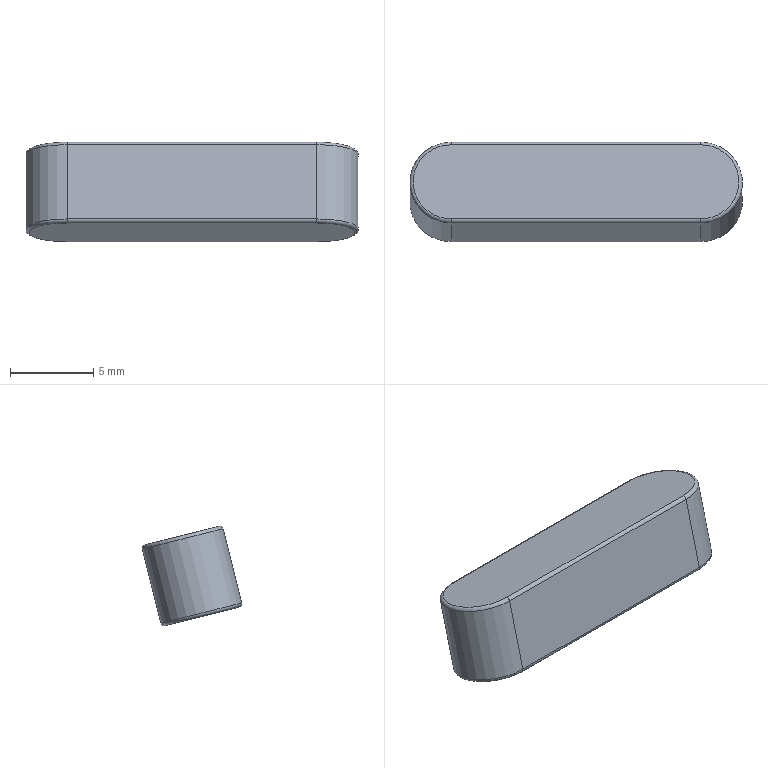Component | NX | STANDARD_FLAT_KEY_A_5X5X20 | 1 solid | 14 faces | box 20 x 5.98 x 5.98 mm | volume 472 mm3 | cylinder 6 | plane 4 | torus 4 | commonest cylinder face diameters 0.4 x4 5 x2
STEP:
#1=CARTESIAN_POINT('',(0.,0.,0.));
#2=DIRECTION('',(0.,0.,1.));
#3=DIRECTION('',(1.,0.,0.));
#4=AXIS2_PLACEMENT_3D('',#1,#2,#3);
#5=CARTESIAN_POINT('',(-38.948,64.186,69.841));
#6=VERTEX_POINT('',#5);
#7=CARTESIAN_POINT('',(-38.948,63.064,65.38));
#8=VERTEX_POINT('',#7);
#9=CARTESIAN_POINT('',(-38.948,64.235,70.035));
#10=DIRECTION('',(0.,-0.2438,-0.9698));
#11=VECTOR('',#10,1.);
#12=LINE('',#9,#11);
#13=CARTESIAN_POINT('',(-38.948,66.659,69.426));
#14=DIRECTION('',(0.,-0.2438,-0.9698));
#15=DIRECTION('',(1.,0.,0.));
#16=AXIS2_PLACEMENT_3D('',#13,#14,#15);
#17=CYLINDRICAL_SURFACE('',#16,2.5);
#18=CARTESIAN_POINT('',(1.571,0.));
#19=DIRECTION('',(0.,1.));
#20=VECTOR('',#19,1.);
#21=LINE('',#18,#20);
#22=(GEOMETRIC_REPRESENTATION_CONTEXT(2)PARAMETRIC_REPRESENTATION_CONTEXT()REPRESENTATION_CONTEXT('',''));
#23=DEFINITIONAL_REPRESENTATION('',(#21),#22);
#24=PCURVE('',#17,#23);
#25=CARTESIAN_POINT('',(-23.948,64.235,70.035));
#26=DIRECTION('',(-0.,-0.9698,0.2438));
#27=DIRECTION('',(-1.,0.,-0.));
#28=AXIS2_PLACEMENT_3D('',#25,#26,#27);
#29=PLANE('',#28);
#30=CARTESIAN_POINT('',(15.,-0.));
#31=DIRECTION('',(-0.,1.));
#32=VECTOR('',#31,1.);
#33=LINE('',#30,#32);
#34=(GEOMETRIC_REPRESENTATION_CONTEXT(2)PARAMETRIC_REPRESENTATION_CONTEXT()REPRESENTATION_CONTEXT('',''));
#35=DEFINITIONAL_REPRESENTATION('',(#33),#34);
#36=PCURVE('',#29,#35);
#37=SURFACE_CURVE('',#12,(#24,#36),.PCURVE_S1.);
#38=EDGE_CURVE('',#6,#8,#37,.T.);
#39=ORIENTED_EDGE('',*,*,#38,.F.);
#40=CARTESIAN_POINT('',(-38.948,69.035,68.622));
#41=VERTEX_POINT('',#40);
#42=CARTESIAN_POINT('',(-38.948,66.61,69.232));
#43=DIRECTION('',(0.,-0.2438,-0.9698));
#44=DIRECTION('',(1.,0.,0.));
#45=AXIS2_PLACEMENT_3D('',#42,#43,#44);
#46=CIRCLE('',#45,2.5);
#47=CARTESIAN_POINT('',(0.,0.2));
#48=DIRECTION('',(1.,-0.));
#49=VECTOR('',#48,1.);
#50=LINE('',#47,#49);
#51=(GEOMETRIC_REPRESENTATION_CONTEXT(2)PARAMETRIC_REPRESENTATION_CONTEXT()REPRESENTATION_CONTEXT('',''));
#52=DEFINITIONAL_REPRESENTATION('',(#50),#51);
#53=PCURVE('',#17,#52);
#54=CARTESIAN_POINT('',(-38.948,66.61,69.232));
#55=DIRECTION('',(0.,-0.2438,-0.9698));
#56=DIRECTION('',(1.,0.,0.));
#57=AXIS2_PLACEMENT_3D('',#54,#55,#56);
#58=TOROIDAL_SURFACE('',#57,2.3,0.2);
#59=CARTESIAN_POINT('',(0.,6.283));
#60=DIRECTION('',(1.,0.));
#61=VECTOR('',#60,1.);
#62=LINE('',#59,#61);
#63=(GEOMETRIC_REPRESENTATION_CONTEXT(2)PARAMETRIC_REPRESENTATION_CONTEXT()REPRESENTATION_CONTEXT('',''));
#64=DEFINITIONAL_REPRESENTATION('',(#62),#63);
#65=PCURVE('',#58,#64);
#66=SURFACE_CURVE('',#46,(#53,#65),.PCURVE_S1.);
#67=EDGE_CURVE('',#6,#41,#66,.T.);
#68=ORIENTED_EDGE('',*,*,#67,.T.);
#69=CARTESIAN_POINT('',(-38.948,67.914,64.161));
#70=VERTEX_POINT('',#69);
#71=CARTESIAN_POINT('',(-38.948,69.084,68.816));
#72=DIRECTION('',(0.,-0.2438,-0.9698));
#73=VECTOR('',#72,1.);
#74=LINE('',#71,#73);
#75=CARTESIAN_POINT('',(4.712,0.));
#76=DIRECTION('',(0.,1.));
#77=VECTOR('',#76,1.);
#78=LINE('',#75,#77);
#79=(GEOMETRIC_REPRESENTATION_CONTEXT(2)PARAMETRIC_REPRESENTATION_CONTEXT()REPRESENTATION_CONTEXT('',''));
#80=DEFINITIONAL_REPRESENTATION('',(#78),#79);
#81=PCURVE('',#17,#80);
#82=CARTESIAN_POINT('',(-38.948,69.084,68.816));
#83=DIRECTION('',(0.,0.9698,-0.2438));
#84=DIRECTION('',(0.,0.2438,0.9698));
#85=AXIS2_PLACEMENT_3D('',#82,#83,#84);
#86=PLANE('',#85);
#87=CARTESIAN_POINT('',(0.,0.));
#88=DIRECTION('',(-1.,0.));
#89=VECTOR('',#88,1.);
#90=LINE('',#87,#89);
#91=(GEOMETRIC_REPRESENTATION_CONTEXT(2)PARAMETRIC_REPRESENTATION_CONTEXT()REPRESENTATION_CONTEXT('',''));
#92=DEFINITIONAL_REPRESENTATION('',(#90),#91);
#93=PCURVE('',#86,#92);
#94=SURFACE_CURVE('',#74,(#81,#93),.PCURVE_S1.);
#95=EDGE_CURVE('',#41,#70,#94,.T.);
#96=ORIENTED_EDGE('',*,*,#95,.T.);
#97=CARTESIAN_POINT('',(-38.948,65.489,64.77));
#98=DIRECTION('',(0.,0.2438,0.9698));
#99=DIRECTION('',(1.,0.,0.));
#100=AXIS2_PLACEMENT_3D('',#97,#98,#99);
#101=CIRCLE('',#100,2.5);
#102=CARTESIAN_POINT('',(6.283,4.8));
#103=DIRECTION('',(-1.,0.));
#104=VECTOR('',#103,1.);
#105=LINE('',#102,#104);
#106=(GEOMETRIC_REPRESENTATION_CONTEXT(2)PARAMETRIC_REPRESENTATION_CONTEXT()REPRESENTATION_CONTEXT('',''));
#107=DEFINITIONAL_REPRESENTATION('',(#105),#106);
#108=PCURVE('',#17,#107);
#109=CARTESIAN_POINT('',(-38.948,65.489,64.77));
#110=DIRECTION('',(0.,-0.2438,-0.9698));
#111=DIRECTION('',(1.,0.,0.));
#112=AXIS2_PLACEMENT_3D('',#109,#110,#111);
#113=TOROIDAL_SURFACE('',#112,2.3,0.2);
#114=CARTESIAN_POINT('',(6.283,0.));
#115=DIRECTION('',(-1.,0.));
#116=VECTOR('',#115,1.);
#117=LINE('',#114,#116);
#118=(GEOMETRIC_REPRESENTATION_CONTEXT(2)PARAMETRIC_REPRESENTATION_CONTEXT()REPRESENTATION_CONTEXT('',''));
#119=DEFINITIONAL_REPRESENTATION('',(#117),#118);
#120=PCURVE('',#113,#119);
#121=SURFACE_CURVE('',#101,(#108,#120),.PCURVE_S1.);
#122=EDGE_CURVE('',#70,#8,#121,.T.);
#123=ORIENTED_EDGE('',*,*,#122,.T.);
#124=EDGE_LOOP('',(#39,#68,#96,#123));
#125=FACE_BOUND('',#124,.T.);
#126=ADVANCED_FACE('',(#125),#17,.T.);
#127=ORIENTED_EDGE('',*,*,#95,.F.);
#128=CARTESIAN_POINT('',(-23.948,69.035,68.622));
#129=VERTEX_POINT('',#128);
#130=CARTESIAN_POINT('',(-23.948,69.035,68.622));
#131=DIRECTION('',(1.,0.,0.));
#132=VECTOR('',#131,1.);
#133=LINE('',#130,#132);
#134=CARTESIAN_POINT('',(-0.2,15.));
#135=DIRECTION('',(0.,1.));
#136=VECTOR('',#135,1.);
#137=LINE('',#134,#136);
#138=(GEOMETRIC_REPRESENTATION_CONTEXT(2)PARAMETRIC_REPRESENTATION_CONTEXT()REPRESENTATION_CONTEXT('',''));
#139=DEFINITIONAL_REPRESENTATION('',(#137),#138);
#140=PCURVE('',#86,#139);
#141=CARTESIAN_POINT('',(-38.948,68.841,68.671));
#142=DIRECTION('',(-1.,0.,0.));
#143=DIRECTION('',(0.,-0.2438,-0.9698));
#144=AXIS2_PLACEMENT_3D('',#141,#142,#143);
#145=CYLINDRICAL_SURFACE('',#144,0.2);
#146=CARTESIAN_POINT('',(4.712,-15.));
#147=DIRECTION('',(0.,-1.));
#148=VECTOR('',#147,1.);
#149=LINE('',#146,#148);
#150=(GEOMETRIC_REPRESENTATION_CONTEXT(2)PARAMETRIC_REPRESENTATION_CONTEXT()REPRESENTATION_CONTEXT('',''));
#151=DEFINITIONAL_REPRESENTATION('',(#149),#150);
#152=PCURVE('',#145,#151);
#153=SURFACE_CURVE('',#133,(#140,#152),.PCURVE_S1.);
#154=EDGE_CURVE('',#41,#129,#153,.T.);
#155=ORIENTED_EDGE('',*,*,#154,.T.);
#156=CARTESIAN_POINT('',(-23.948,67.914,64.161));
#157=VERTEX_POINT('',#156);
#158=CARTESIAN_POINT('',(-23.948,69.084,68.816));
#159=DIRECTION('',(0.,-0.2438,-0.9698));
#160=VECTOR('',#159,1.);
#161=LINE('',#158,#160);
#162=CARTESIAN_POINT('',(0.,15.));
#163=DIRECTION('',(-1.,0.));
#164=VECTOR('',#163,1.);
#165=LINE('',#162,#164);
#166=(GEOMETRIC_REPRESENTATION_CONTEXT(2)PARAMETRIC_REPRESENTATION_CONTEXT()REPRESENTATION_CONTEXT('',''));
#167=DEFINITIONAL_REPRESENTATION('',(#165),#166);
#168=PCURVE('',#86,#167);
#169=CARTESIAN_POINT('',(-23.948,66.659,69.426));
#170=DIRECTION('',(0.,-0.2438,-0.9698));
#171=DIRECTION('',(1.,0.,0.));
#172=AXIS2_PLACEMENT_3D('',#169,#170,#171);
#173=CYLINDRICAL_SURFACE('',#172,2.5);
#174=CARTESIAN_POINT('',(4.712,0.));
#175=DIRECTION('',(0.,1.));
#176=VECTOR('',#175,1.);
#177=LINE('',#174,#176);
#178=(GEOMETRIC_REPRESENTATION_CONTEXT(2)PARAMETRIC_REPRESENTATION_CONTEXT()REPRESENTATION_CONTEXT('',''));
#179=DEFINITIONAL_REPRESENTATION('',(#177),#178);
#180=PCURVE('',#173,#179);
#181=SURFACE_CURVE('',#161,(#168,#180),.PCURVE_S1.);
#182=EDGE_CURVE('',#129,#157,#181,.T.);
#183=ORIENTED_EDGE('',*,*,#182,.T.);
#184=CARTESIAN_POINT('',(-38.948,67.914,64.161));
#185=DIRECTION('',(-1.,0.,0.));
#186=VECTOR('',#185,1.);
#187=LINE('',#184,#186);
#188=CARTESIAN_POINT('',(-4.8,0.));
#189=DIRECTION('',(0.,-1.));
#190=VECTOR('',#189,1.);
#191=LINE('',#188,#190);
#192=(GEOMETRIC_REPRESENTATION_CONTEXT(2)PARAMETRIC_REPRESENTATION_CONTEXT()REPRESENTATION_CONTEXT('',''));
#193=DEFINITIONAL_REPRESENTATION('',(#191),#192);
#194=PCURVE('',#86,#193);
#195=CARTESIAN_POINT('',(-38.948,67.72,64.21));
#196=DIRECTION('',(1.,0.,0.));
#197=DIRECTION('',(0.,0.2438,0.9698));
#198=AXIS2_PLACEMENT_3D('',#195,#196,#197);
#199=CYLINDRICAL_SURFACE('',#198,0.2);
#200=CARTESIAN_POINT('',(4.712,0.));
#201=DIRECTION('',(0.,-1.));
#202=VECTOR('',#201,1.);
#203=LINE('',#200,#202);
#204=(GEOMETRIC_REPRESENTATION_CONTEXT(2)PARAMETRIC_REPRESENTATION_CONTEXT()REPRESENTATION_CONTEXT('',''));
#205=DEFINITIONAL_REPRESENTATION('',(#203),#204);
#206=PCURVE('',#199,#205);
#207=SURFACE_CURVE('',#187,(#194,#206),.PCURVE_S1.);
#208=EDGE_CURVE('',#157,#70,#207,.T.);
#209=ORIENTED_EDGE('',*,*,#208,.T.);
#210=EDGE_LOOP('',(#127,#155,#183,#209));
#211=FACE_BOUND('',#210,.T.);
#212=ADVANCED_FACE('',(#211),#86,.T.);
#213=ORIENTED_EDGE('',*,*,#182,.F.);
#214=CARTESIAN_POINT('',(-23.948,64.186,69.841));
#215=VERTEX_POINT('',#214);
#216=CARTESIAN_POINT('',(-23.948,66.61,69.232));
#217=DIRECTION('',(0.,-0.2438,-0.9698));
#218=DIRECTION('',(1.,0.,0.));
#219=AXIS2_PLACEMENT_3D('',#216,#217,#218);
#220=CIRCLE('',#219,2.5);
#221=CARTESIAN_POINT('',(0.,0.2));
#222=DIRECTION('',(1.,0.));
#223=VECTOR('',#222,1.);
#224=LINE('',#221,#223);
#225=(GEOMETRIC_REPRESENTATION_CONTEXT(2)PARAMETRIC_REPRESENTATION_CONTEXT()REPRESENTATION_CONTEXT('',''));
#226=DEFINITIONAL_REPRESENTATION('',(#224),#225);
#227=PCURVE('',#173,#226);
#228=CARTESIAN_POINT('',(-23.948,66.61,69.232));
#229=DIRECTION('',(0.,-0.2438,-0.9698));
#230=DIRECTION('',(1.,0.,0.));
#231=AXIS2_PLACEMENT_3D('',#228,#229,#230);
#232=TOROIDAL_SURFACE('',#231,2.3,0.2);
#233=CARTESIAN_POINT('',(-0.,6.283));
#234=DIRECTION('',(1.,0.));
#235=VECTOR('',#234,1.);
#236=LINE('',#233,#235);
#237=(GEOMETRIC_REPRESENTATION_CONTEXT(2)PARAMETRIC_REPRESENTATION_CONTEXT()REPRESENTATION_CONTEXT('',''));
#238=DEFINITIONAL_REPRESENTATION('',(#236),#237);
#239=PCURVE('',#232,#238);
#240=SURFACE_CURVE('',#220,(#227,#239),.PCURVE_S1.);
#241=EDGE_CURVE('',#129,#215,#240,.T.);
#242=ORIENTED_EDGE('',*,*,#241,.T.);
#243=CARTESIAN_POINT('',(-23.948,63.064,65.38));
#244=VERTEX_POINT('',#243);
#245=CARTESIAN_POINT('',(-23.948,64.235,70.035));
#246=DIRECTION('',(0.,-0.2438,-0.9698));
#247=VECTOR('',#246,1.);
#248=LINE('',#245,#247);
#249=CARTESIAN_POINT('',(7.854,-0.));
#250=DIRECTION('',(0.,1.));
#251=VECTOR('',#250,1.);
#252=LINE('',#249,#251);
#253=(GEOMETRIC_REPRESENTATION_CONTEXT(2)PARAMETRIC_REPRESENTATION_CONTEXT()REPRESENTATION_CONTEXT('',''));
#254=DEFINITIONAL_REPRESENTATION('',(#252),#253);
#255=PCURVE('',#173,#254);
#256=CARTESIAN_POINT('',(-0.,-0.));
#257=DIRECTION('',(-0.,1.));
#258=VECTOR('',#257,1.);
#259=LINE('',#256,#258);
#260=(GEOMETRIC_REPRESENTATION_CONTEXT(2)PARAMETRIC_REPRESENTATION_CONTEXT()REPRESENTATION_CONTEXT('',''));
#261=DEFINITIONAL_REPRESENTATION('',(#259),#260);
#262=PCURVE('',#29,#261);
#263=SURFACE_CURVE('',#248,(#255,#262),.PCURVE_S1.);
#264=EDGE_CURVE('',#215,#244,#263,.T.);
#265=ORIENTED_EDGE('',*,*,#264,.T.);
#266=CARTESIAN_POINT('',(-23.948,65.489,64.77));
#267=DIRECTION('',(0.,0.2438,0.9698));
#268=DIRECTION('',(1.,0.,0.));
#269=AXIS2_PLACEMENT_3D('',#266,#267,#268);
#270=CIRCLE('',#269,2.5);
#271=CARTESIAN_POINT('',(12.566,4.8));
#272=DIRECTION('',(-1.,0.));
#273=VECTOR('',#272,1.);
#274=LINE('',#271,#273);
#275=(GEOMETRIC_REPRESENTATION_CONTEXT(2)PARAMETRIC_REPRESENTATION_CONTEXT()REPRESENTATION_CONTEXT('',''));
#276=DEFINITIONAL_REPRESENTATION('',(#274),#275);
#277=PCURVE('',#173,#276);
#278=CARTESIAN_POINT('',(-23.948,65.489,64.77));
#279=DIRECTION('',(0.,-0.2438,-0.9698));
#280=DIRECTION('',(1.,0.,0.));
#281=AXIS2_PLACEMENT_3D('',#278,#279,#280);
#282=TOROIDAL_SURFACE('',#281,2.3,0.2);
#283=CARTESIAN_POINT('',(12.566,0.));
#284=DIRECTION('',(-1.,0.));
#285=VECTOR('',#284,1.);
#286=LINE('',#283,#285);
#287=(GEOMETRIC_REPRESENTATION_CONTEXT(2)PARAMETRIC_REPRESENTATION_CONTEXT()REPRESENTATION_CONTEXT('',''));
#288=DEFINITIONAL_REPRESENTATION('',(#286),#287);
#289=PCURVE('',#282,#288);
#290=SURFACE_CURVE('',#270,(#277,#289),.PCURVE_S1.);
#291=EDGE_CURVE('',#244,#157,#290,.T.);
#292=ORIENTED_EDGE('',*,*,#291,.T.);
#293=EDGE_LOOP('',(#213,#242,#265,#292));
#294=FACE_BOUND('',#293,.T.);
#295=ADVANCED_FACE('',(#294),#173,.T.);
#296=ORIENTED_EDGE('',*,*,#264,.F.);
#297=CARTESIAN_POINT('',(-38.948,64.186,69.841));
#298=DIRECTION('',(-1.,0.,-0.));
#299=VECTOR('',#298,1.);
#300=LINE('',#297,#299);
#301=CARTESIAN_POINT('',(15.,0.2));
#302=DIRECTION('',(1.,0.));
#303=VECTOR('',#302,1.);
#304=LINE('',#301,#303);
#305=(GEOMETRIC_REPRESENTATION_CONTEXT(2)PARAMETRIC_REPRESENTATION_CONTEXT()REPRESENTATION_CONTEXT('',''));
#306=DEFINITIONAL_REPRESENTATION('',(#304),#305);
#307=PCURVE('',#29,#306);
#308=CARTESIAN_POINT('',(-23.948,64.38,69.792));
#309=DIRECTION('',(1.,-0.,0.));
#310=DIRECTION('',(-0.,-0.9698,0.2438));
#311=AXIS2_PLACEMENT_3D('',#308,#309,#310);
#312=CYLINDRICAL_SURFACE('',#311,0.2);
#313=CARTESIAN_POINT('',(6.283,-15.));
#314=DIRECTION('',(0.,-1.));
#315=VECTOR('',#314,1.);
#316=LINE('',#313,#315);
#317=(GEOMETRIC_REPRESENTATION_CONTEXT(2)PARAMETRIC_REPRESENTATION_CONTEXT()REPRESENTATION_CONTEXT('',''));
#318=DEFINITIONAL_REPRESENTATION('',(#316),#317);
#319=PCURVE('',#312,#318);
#320=SURFACE_CURVE('',#300,(#307,#319),.PCURVE_S1.);
#321=EDGE_CURVE('',#215,#6,#320,.T.);
#322=ORIENTED_EDGE('',*,*,#321,.T.);
#323=ORIENTED_EDGE('',*,*,#38,.T.);
#324=CARTESIAN_POINT('',(-23.948,63.064,65.38));
#325=DIRECTION('',(1.,-0.,0.));
#326=VECTOR('',#325,1.);
#327=LINE('',#324,#326);
#328=CARTESIAN_POINT('',(-0.,4.8));
#329=DIRECTION('',(-1.,-0.));
#330=VECTOR('',#329,1.);
#331=LINE('',#328,#330);
#332=(GEOMETRIC_REPRESENTATION_CONTEXT(2)PARAMETRIC_REPRESENTATION_CONTEXT()REPRESENTATION_CONTEXT('',''));
#333=DEFINITIONAL_REPRESENTATION('',(#331),#332);
#334=PCURVE('',#29,#333);
#335=CARTESIAN_POINT('',(-38.948,63.258,65.331));
#336=DIRECTION('',(-1.,0.,-0.));
#337=DIRECTION('',(0.,0.9698,-0.2438));
#338=AXIS2_PLACEMENT_3D('',#335,#336,#337);
#339=CYLINDRICAL_SURFACE('',#338,0.2);
#340=CARTESIAN_POINT('',(3.142,-15.));
#341=DIRECTION('',(0.,-1.));
#342=VECTOR('',#341,1.);
#343=LINE('',#340,#342);
#344=(GEOMETRIC_REPRESENTATION_CONTEXT(2)PARAMETRIC_REPRESENTATION_CONTEXT()REPRESENTATION_CONTEXT('',''));
#345=DEFINITIONAL_REPRESENTATION('',(#343),#344);
#346=PCURVE('',#339,#345);
#347=SURFACE_CURVE('',#327,(#334,#346),.PCURVE_S1.);
#348=EDGE_CURVE('',#8,#244,#347,.T.);
#349=ORIENTED_EDGE('',*,*,#348,.T.);
#350=EDGE_LOOP('',(#296,#322,#323,#349));
#351=FACE_BOUND('',#350,.T.);
#352=ADVANCED_FACE('',(#351),#29,.T.);
#353=CARTESIAN_POINT('',(-38.948,68.89,68.865));
#354=VERTEX_POINT('',#353);
#355=CARTESIAN_POINT('',(-38.948,64.429,69.986));
#356=VERTEX_POINT('',#355);
#357=CARTESIAN_POINT('',(-38.948,66.659,69.426));
#358=DIRECTION('',(0.,0.2438,0.9698));
#359=DIRECTION('',(1.,0.,0.));
#360=AXIS2_PLACEMENT_3D('',#357,#358,#359);
#361=CIRCLE('',#360,2.3);
#362=CARTESIAN_POINT('',(-38.948,66.659,69.426));
#363=DIRECTION('',(0.,-0.2438,-0.9698));
#364=DIRECTION('',(1.,0.,0.));
#365=AXIS2_PLACEMENT_3D('',#362,#363,#364);
#366=PLANE('',#365);
#367=CARTESIAN_POINT('',(2.3,0.));
#368=CARTESIAN_POINT('',(2.3,-3.984));
#369=CARTESIAN_POINT('',(-1.15,-1.992));
#370=CARTESIAN_POINT('',(-4.6,-0.));
#371=CARTESIAN_POINT('',(-1.15,1.992));
#372=CARTESIAN_POINT('',(2.3,3.984));
#373=CARTESIAN_POINT('',(2.3,0.));
#374=(BOUNDED_CURVE()B_SPLINE_CURVE(2,(#367,#368,#369,#370,#371,#372,#373),.UNSPECIFIED.,.T.,.F.)B_SPLINE_CURVE_WITH_KNOTS((1,2,2,2,2,1),(-2.094,0.,2.094,4.189,6.283,8.378),.UNSPECIFIED.)CURVE()GEOMETRIC_REPRESENTATION_ITEM()RATIONAL_B_SPLINE_CURVE((1.,0.5,1.,0.5,1.,0.5,1.))REPRESENTATION_ITEM(''));
#375=(GEOMETRIC_REPRESENTATION_CONTEXT(2)PARAMETRIC_REPRESENTATION_CONTEXT()REPRESENTATION_CONTEXT('',''));
#376=DEFINITIONAL_REPRESENTATION('',(#374),#375);
#377=PCURVE('',#366,#376);
#378=CARTESIAN_POINT('',(6.283,4.712));
#379=DIRECTION('',(-1.,0.));
#380=VECTOR('',#379,1.);
#381=LINE('',#378,#380);
#382=(GEOMETRIC_REPRESENTATION_CONTEXT(2)PARAMETRIC_REPRESENTATION_CONTEXT()REPRESENTATION_CONTEXT('',''));
#383=DEFINITIONAL_REPRESENTATION('',(#381),#382);
#384=PCURVE('',#58,#383);
#385=SURFACE_CURVE('',#361,(#377,#384),.PCURVE_S1.);
#386=EDGE_CURVE('',#354,#356,#385,.T.);
#387=ORIENTED_EDGE('',*,*,#386,.T.);
#388=CARTESIAN_POINT('',(-23.948,64.429,69.986));
#389=VERTEX_POINT('',#388);
#390=CARTESIAN_POINT('',(-23.948,64.429,69.986));
#391=DIRECTION('',(1.,-0.,0.));
#392=VECTOR('',#391,1.);
#393=LINE('',#390,#392);
#394=CARTESIAN_POINT('',(15.,2.3));
#395=DIRECTION('',(1.,0.));
#396=VECTOR('',#395,1.);
#397=LINE('',#394,#396);
#398=(GEOMETRIC_REPRESENTATION_CONTEXT(2)PARAMETRIC_REPRESENTATION_CONTEXT()REPRESENTATION_CONTEXT('',''));
#399=DEFINITIONAL_REPRESENTATION('',(#397),#398);
#400=PCURVE('',#366,#399);
#401=CARTESIAN_POINT('',(4.712,0.));
#402=DIRECTION('',(0.,1.));
#403=VECTOR('',#402,1.);
#404=LINE('',#401,#403);
#405=(GEOMETRIC_REPRESENTATION_CONTEXT(2)PARAMETRIC_REPRESENTATION_CONTEXT()REPRESENTATION_CONTEXT('',''));
#406=DEFINITIONAL_REPRESENTATION('',(#404),#405);
#407=PCURVE('',#312,#406);
#408=SURFACE_CURVE('',#393,(#400,#407),.PCURVE_S1.);
#409=EDGE_CURVE('',#356,#389,#408,.T.);
#410=ORIENTED_EDGE('',*,*,#409,.T.);
#411=CARTESIAN_POINT('',(-23.948,68.89,68.865));
#412=VERTEX_POINT('',#411);
#413=CARTESIAN_POINT('',(-23.948,66.659,69.426));
#414=DIRECTION('',(0.,0.2438,0.9698));
#415=DIRECTION('',(1.,0.,0.));
#416=AXIS2_PLACEMENT_3D('',#413,#414,#415);
#417=CIRCLE('',#416,2.3);
#418=CARTESIAN_POINT('',(17.3,0.));
#419=CARTESIAN_POINT('',(17.3,-3.984));
#420=CARTESIAN_POINT('',(13.85,-1.992));
#421=CARTESIAN_POINT('',(10.4,-0.));
#422=CARTESIAN_POINT('',(13.85,1.992));
#423=CARTESIAN_POINT('',(17.3,3.984));
#424=CARTESIAN_POINT('',(17.3,0.));
#425=(BOUNDED_CURVE()B_SPLINE_CURVE(2,(#418,#419,#420,#421,#422,#423,#424),.UNSPECIFIED.,.T.,.F.)B_SPLINE_CURVE_WITH_KNOTS((1,2,2,2,2,1),(-2.094,0.,2.094,4.189,6.283,8.378),.UNSPECIFIED.)CURVE()GEOMETRIC_REPRESENTATION_ITEM()RATIONAL_B_SPLINE_CURVE((1.,0.5,1.,0.5,1.,0.5,1.))REPRESENTATION_ITEM(''));
#426=(GEOMETRIC_REPRESENTATION_CONTEXT(2)PARAMETRIC_REPRESENTATION_CONTEXT()REPRESENTATION_CONTEXT('',''));
#427=DEFINITIONAL_REPRESENTATION('',(#425),#426);
#428=PCURVE('',#366,#427);
#429=CARTESIAN_POINT('',(12.566,4.712));
#430=DIRECTION('',(-1.,-0.));
#431=VECTOR('',#430,1.);
#432=LINE('',#429,#431);
#433=(GEOMETRIC_REPRESENTATION_CONTEXT(2)PARAMETRIC_REPRESENTATION_CONTEXT()REPRESENTATION_CONTEXT('',''));
#434=DEFINITIONAL_REPRESENTATION('',(#432),#433);
#435=PCURVE('',#232,#434);
#436=SURFACE_CURVE('',#417,(#428,#435),.PCURVE_S1.);
#437=EDGE_CURVE('',#389,#412,#436,.T.);
#438=ORIENTED_EDGE('',*,*,#437,.T.);
#439=CARTESIAN_POINT('',(-38.948,68.89,68.865));
#440=DIRECTION('',(-1.,0.,0.));
#441=VECTOR('',#440,1.);
#442=LINE('',#439,#441);
#443=CARTESIAN_POINT('',(0.,-2.3));
#444=DIRECTION('',(-1.,0.));
#445=VECTOR('',#444,1.);
#446=LINE('',#443,#445);
#447=(GEOMETRIC_REPRESENTATION_CONTEXT(2)PARAMETRIC_REPRESENTATION_CONTEXT()REPRESENTATION_CONTEXT('',''));
#448=DEFINITIONAL_REPRESENTATION('',(#446),#447);
#449=PCURVE('',#366,#448);
#450=CARTESIAN_POINT('',(3.142,0.));
#451=DIRECTION('',(0.,1.));
#452=VECTOR('',#451,1.);
#453=LINE('',#450,#452);
#454=(GEOMETRIC_REPRESENTATION_CONTEXT(2)PARAMETRIC_REPRESENTATION_CONTEXT()REPRESENTATION_CONTEXT('',''));
#455=DEFINITIONAL_REPRESENTATION('',(#453),#454);
#456=PCURVE('',#145,#455);
#457=SURFACE_CURVE('',#442,(#449,#456),.PCURVE_S1.);
#458=EDGE_CURVE('',#412,#354,#457,.T.);
#459=ORIENTED_EDGE('',*,*,#458,.T.);
#460=EDGE_LOOP('',(#387,#410,#438,#459));
#461=FACE_BOUND('',#460,.T.);
#462=ADVANCED_FACE('',(#461),#366,.F.);
#463=CARTESIAN_POINT('',(-23.948,67.671,64.016));
#464=VERTEX_POINT('',#463);
#465=CARTESIAN_POINT('',(-23.948,63.21,65.137));
#466=VERTEX_POINT('',#465);
#467=CARTESIAN_POINT('',(-23.948,65.44,64.577));
#468=DIRECTION('',(0.,-0.2438,-0.9698));
#469=DIRECTION('',(1.,0.,0.));
#470=AXIS2_PLACEMENT_3D('',#467,#468,#469);
#471=CIRCLE('',#470,2.3);
#472=CARTESIAN_POINT('',(-38.948,65.44,64.577));
#473=DIRECTION('',(0.,-0.2438,-0.9698));
#474=DIRECTION('',(1.,0.,0.));
#475=AXIS2_PLACEMENT_3D('',#472,#473,#474);
#476=PLANE('',#475);
#477=CARTESIAN_POINT('',(15.,0.));
#478=DIRECTION('',(1.,0.));
#479=AXIS2_PLACEMENT_2D('',#477,#478);
#480=CIRCLE('',#479,2.3);
#481=(GEOMETRIC_REPRESENTATION_CONTEXT(2)PARAMETRIC_REPRESENTATION_CONTEXT()REPRESENTATION_CONTEXT('',''));
#482=DEFINITIONAL_REPRESENTATION('',(#480),#481);
#483=PCURVE('',#476,#482);
#484=CARTESIAN_POINT('',(0.,1.571));
#485=DIRECTION('',(1.,-0.));
#486=VECTOR('',#485,1.);
#487=LINE('',#484,#486);
#488=(GEOMETRIC_REPRESENTATION_CONTEXT(2)PARAMETRIC_REPRESENTATION_CONTEXT()REPRESENTATION_CONTEXT('',''));
#489=DEFINITIONAL_REPRESENTATION('',(#487),#488);
#490=PCURVE('',#282,#489);
#491=SURFACE_CURVE('',#471,(#483,#490),.PCURVE_S1.);
#492=EDGE_CURVE('',#464,#466,#491,.T.);
#493=ORIENTED_EDGE('',*,*,#492,.T.);
#494=CARTESIAN_POINT('',(-38.948,63.21,65.137));
#495=VERTEX_POINT('',#494);
#496=CARTESIAN_POINT('',(-38.948,63.21,65.137));
#497=DIRECTION('',(-1.,0.,-0.));
#498=VECTOR('',#497,1.);
#499=LINE('',#496,#498);
#500=CARTESIAN_POINT('',(0.,2.3));
#501=DIRECTION('',(-1.,-0.));
#502=VECTOR('',#501,1.);
#503=LINE('',#500,#502);
#504=(GEOMETRIC_REPRESENTATION_CONTEXT(2)PARAMETRIC_REPRESENTATION_CONTEXT()REPRESENTATION_CONTEXT('',''));
#505=DEFINITIONAL_REPRESENTATION('',(#503),#504);
#506=PCURVE('',#476,#505);
#507=CARTESIAN_POINT('',(1.571,0.));
#508=DIRECTION('',(0.,1.));
#509=VECTOR('',#508,1.);
#510=LINE('',#507,#509);
#511=(GEOMETRIC_REPRESENTATION_CONTEXT(2)PARAMETRIC_REPRESENTATION_CONTEXT()REPRESENTATION_CONTEXT('',''));
#512=DEFINITIONAL_REPRESENTATION('',(#510),#511);
#513=PCURVE('',#339,#512);
#514=SURFACE_CURVE('',#499,(#506,#513),.PCURVE_S1.);
#515=EDGE_CURVE('',#466,#495,#514,.T.);
#516=ORIENTED_EDGE('',*,*,#515,.T.);
#517=CARTESIAN_POINT('',(-38.948,67.671,64.016));
#518=VERTEX_POINT('',#517);
#519=CARTESIAN_POINT('',(-38.948,65.44,64.577));
#520=DIRECTION('',(0.,-0.2438,-0.9698));
#521=DIRECTION('',(1.,0.,0.));
#522=AXIS2_PLACEMENT_3D('',#519,#520,#521);
#523=CIRCLE('',#522,2.3);
#524=CARTESIAN_POINT('',(0.,0.));
#525=DIRECTION('',(1.,0.));
#526=AXIS2_PLACEMENT_2D('',#524,#525);
#527=CIRCLE('',#526,2.3);
#528=(GEOMETRIC_REPRESENTATION_CONTEXT(2)PARAMETRIC_REPRESENTATION_CONTEXT()REPRESENTATION_CONTEXT('',''));
#529=DEFINITIONAL_REPRESENTATION('',(#527),#528);
#530=PCURVE('',#476,#529);
#531=CARTESIAN_POINT('',(0.,1.571));
#532=DIRECTION('',(1.,0.));
#533=VECTOR('',#532,1.);
#534=LINE('',#531,#533);
#535=(GEOMETRIC_REPRESENTATION_CONTEXT(2)PARAMETRIC_REPRESENTATION_CONTEXT()REPRESENTATION_CONTEXT('',''));
#536=DEFINITIONAL_REPRESENTATION('',(#534),#535);
#537=PCURVE('',#113,#536);
#538=SURFACE_CURVE('',#523,(#530,#537),.PCURVE_S1.);
#539=EDGE_CURVE('',#495,#518,#538,.T.);
#540=ORIENTED_EDGE('',*,*,#539,.T.);
#541=CARTESIAN_POINT('',(-38.948,67.671,64.016));
#542=DIRECTION('',(1.,0.,0.));
#543=VECTOR('',#542,1.);
#544=LINE('',#541,#543);
#545=CARTESIAN_POINT('',(0.,-2.3));
#546=DIRECTION('',(1.,0.));
#547=VECTOR('',#546,1.);
#548=LINE('',#545,#547);
#549=(GEOMETRIC_REPRESENTATION_CONTEXT(2)PARAMETRIC_REPRESENTATION_CONTEXT()REPRESENTATION_CONTEXT('',''));
#550=DEFINITIONAL_REPRESENTATION('',(#548),#549);
#551=PCURVE('',#476,#550);
#552=CARTESIAN_POINT('',(3.142,0.));
#553=DIRECTION('',(0.,1.));
#554=VECTOR('',#553,1.);
#555=LINE('',#552,#554);
#556=(GEOMETRIC_REPRESENTATION_CONTEXT(2)PARAMETRIC_REPRESENTATION_CONTEXT()REPRESENTATION_CONTEXT('',''));
#557=DEFINITIONAL_REPRESENTATION('',(#555),#556);
#558=PCURVE('',#199,#557);
#559=SURFACE_CURVE('',#544,(#551,#558),.PCURVE_S1.);
#560=EDGE_CURVE('',#518,#464,#559,.T.);
#561=ORIENTED_EDGE('',*,*,#560,.T.);
#562=EDGE_LOOP('',(#493,#516,#540,#561));
#563=FACE_BOUND('',#562,.T.);
#564=ADVANCED_FACE('',(#563),#476,.T.);
#565=CARTESIAN_POINT('',(-38.948,68.841,68.671));
#566=DIRECTION('',(-1.,0.,0.));
#567=DIRECTION('',(0.,-0.2438,-0.9698));
#568=AXIS2_PLACEMENT_3D('',#565,#566,#567);
#569=CIRCLE('',#568,0.2);
#570=CARTESIAN_POINT('',(0.,0.));
#571=DIRECTION('',(1.,0.));
#572=VECTOR('',#571,1.);
#573=LINE('',#570,#572);
#574=(GEOMETRIC_REPRESENTATION_CONTEXT(2)PARAMETRIC_REPRESENTATION_CONTEXT()REPRESENTATION_CONTEXT('',''));
#575=DEFINITIONAL_REPRESENTATION('',(#573),#574);
#576=PCURVE('',#145,#575);
#577=CARTESIAN_POINT('',(4.712,1.571));
#578=DIRECTION('',(0.,1.));
#579=VECTOR('',#578,1.);
#580=LINE('',#577,#579);
#581=(GEOMETRIC_REPRESENTATION_CONTEXT(2)PARAMETRIC_REPRESENTATION_CONTEXT()REPRESENTATION_CONTEXT('',''));
#582=DEFINITIONAL_REPRESENTATION('',(#580),#581);
#583=PCURVE('',#58,#582);
#584=SURFACE_CURVE('',#569,(#576,#583),.PCURVE_S1.);
#585=EDGE_CURVE('',#354,#41,#584,.T.);
#586=ORIENTED_EDGE('',*,*,#585,.F.);
#587=ORIENTED_EDGE('',*,*,#458,.F.);
#588=CARTESIAN_POINT('',(-23.948,68.841,68.671));
#589=DIRECTION('',(1.,-0.,-0.));
#590=DIRECTION('',(0.,0.2438,0.9698));
#591=AXIS2_PLACEMENT_3D('',#588,#589,#590);
#592=CIRCLE('',#591,0.2);
#593=CARTESIAN_POINT('',(9.425,-15.));
#594=DIRECTION('',(-1.,-0.));
#595=VECTOR('',#594,1.);
#596=LINE('',#593,#595);
#597=(GEOMETRIC_REPRESENTATION_CONTEXT(2)PARAMETRIC_REPRESENTATION_CONTEXT()REPRESENTATION_CONTEXT('',''));
#598=DEFINITIONAL_REPRESENTATION('',(#596),#597);
#599=PCURVE('',#145,#598);
#600=CARTESIAN_POINT('',(4.712,10.996));
#601=DIRECTION('',(-0.,-1.));
#602=VECTOR('',#601,1.);
#603=LINE('',#600,#602);
#604=(GEOMETRIC_REPRESENTATION_CONTEXT(2)PARAMETRIC_REPRESENTATION_CONTEXT()REPRESENTATION_CONTEXT('',''));
#605=DEFINITIONAL_REPRESENTATION('',(#603),#604);
#606=PCURVE('',#232,#605);
#607=SURFACE_CURVE('',#592,(#599,#606),.PCURVE_S1.);
#608=EDGE_CURVE('',#129,#412,#607,.T.);
#609=ORIENTED_EDGE('',*,*,#608,.F.);
#610=ORIENTED_EDGE('',*,*,#154,.F.);
#611=EDGE_LOOP('',(#586,#587,#609,#610));
#612=FACE_BOUND('',#611,.T.);
#613=ADVANCED_FACE('',(#612),#145,.T.);
#614=ORIENTED_EDGE('',*,*,#608,.T.);
#615=ORIENTED_EDGE('',*,*,#437,.F.);
#616=CARTESIAN_POINT('',(-23.948,64.38,69.792));
#617=DIRECTION('',(-1.,0.,0.));
#618=DIRECTION('',(-0.,-0.2438,-0.9698));
#619=AXIS2_PLACEMENT_3D('',#616,#617,#618);
#620=CIRCLE('',#619,0.2);
#621=CARTESIAN_POINT('',(7.854,7.854));
#622=DIRECTION('',(-0.,-1.));
#623=VECTOR('',#622,1.);
#624=LINE('',#621,#623);
#625=(GEOMETRIC_REPRESENTATION_CONTEXT(2)PARAMETRIC_REPRESENTATION_CONTEXT()REPRESENTATION_CONTEXT('',''));
#626=DEFINITIONAL_REPRESENTATION('',(#624),#625);
#627=PCURVE('',#232,#626);
#628=CARTESIAN_POINT('',(7.854,0.));
#629=DIRECTION('',(-1.,0.));
#630=VECTOR('',#629,1.);
#631=LINE('',#628,#630);
#632=(GEOMETRIC_REPRESENTATION_CONTEXT(2)PARAMETRIC_REPRESENTATION_CONTEXT()REPRESENTATION_CONTEXT('',''));
#633=DEFINITIONAL_REPRESENTATION('',(#631),#632);
#634=PCURVE('',#312,#633);
#635=SURFACE_CURVE('',#620,(#627,#634),.PCURVE_S1.);
#636=EDGE_CURVE('',#215,#389,#635,.T.);
#637=ORIENTED_EDGE('',*,*,#636,.F.);
#638=ORIENTED_EDGE('',*,*,#241,.F.);
#639=EDGE_LOOP('',(#614,#615,#637,#638));
#640=FACE_BOUND('',#639,.T.);
#641=ADVANCED_FACE('',(#640),#232,.T.);
#642=ORIENTED_EDGE('',*,*,#585,.T.);
#643=ORIENTED_EDGE('',*,*,#67,.F.);
#644=CARTESIAN_POINT('',(-38.948,64.38,69.792));
#645=DIRECTION('',(1.,-0.,0.));
#646=DIRECTION('',(-0.,-0.9698,0.2438));
#647=AXIS2_PLACEMENT_3D('',#644,#645,#646);
#648=CIRCLE('',#647,0.2);
#649=CARTESIAN_POINT('',(1.571,-0.));
#650=DIRECTION('',(0.,1.));
#651=VECTOR('',#650,1.);
#652=LINE('',#649,#651);
#653=(GEOMETRIC_REPRESENTATION_CONTEXT(2)PARAMETRIC_REPRESENTATION_CONTEXT()REPRESENTATION_CONTEXT('',''));
#654=DEFINITIONAL_REPRESENTATION('',(#652),#653);
#655=PCURVE('',#58,#654);
#656=CARTESIAN_POINT('',(0.,-15.));
#657=DIRECTION('',(1.,0.));
#658=VECTOR('',#657,1.);
#659=LINE('',#656,#658);
#660=(GEOMETRIC_REPRESENTATION_CONTEXT(2)PARAMETRIC_REPRESENTATION_CONTEXT()REPRESENTATION_CONTEXT('',''));
#661=DEFINITIONAL_REPRESENTATION('',(#659),#660);
#662=PCURVE('',#312,#661);
#663=SURFACE_CURVE('',#648,(#655,#662),.PCURVE_S1.);
#664=EDGE_CURVE('',#356,#6,#663,.T.);
#665=ORIENTED_EDGE('',*,*,#664,.F.);
#666=ORIENTED_EDGE('',*,*,#386,.F.);
#667=EDGE_LOOP('',(#642,#643,#665,#666));
#668=FACE_BOUND('',#667,.T.);
#669=ADVANCED_FACE('',(#668),#58,.T.);
#670=ORIENTED_EDGE('',*,*,#636,.T.);
#671=ORIENTED_EDGE('',*,*,#409,.F.);
#672=ORIENTED_EDGE('',*,*,#664,.T.);
#673=ORIENTED_EDGE('',*,*,#321,.F.);
#674=EDGE_LOOP('',(#670,#671,#672,#673));
#675=FACE_BOUND('',#674,.T.);
#676=ADVANCED_FACE('',(#675),#312,.T.);
#677=CARTESIAN_POINT('',(-38.948,67.72,64.21));
#678=DIRECTION('',(-1.,0.,0.));
#679=DIRECTION('',(0.,-0.2438,-0.9698));
#680=AXIS2_PLACEMENT_3D('',#677,#678,#679);
#681=CIRCLE('',#680,0.2);
#682=CARTESIAN_POINT('',(9.425,0.));
#683=DIRECTION('',(-1.,0.));
#684=VECTOR('',#683,1.);
#685=LINE('',#682,#684);
#686=(GEOMETRIC_REPRESENTATION_CONTEXT(2)PARAMETRIC_REPRESENTATION_CONTEXT()REPRESENTATION_CONTEXT('',''));
#687=DEFINITIONAL_REPRESENTATION('',(#685),#686);
#688=PCURVE('',#199,#687);
#689=CARTESIAN_POINT('',(4.712,-4.712));
#690=DIRECTION('',(0.,1.));
#691=VECTOR('',#690,1.);
#692=LINE('',#689,#691);
#693=(GEOMETRIC_REPRESENTATION_CONTEXT(2)PARAMETRIC_REPRESENTATION_CONTEXT()REPRESENTATION_CONTEXT('',''));
#694=DEFINITIONAL_REPRESENTATION('',(#692),#693);
#695=PCURVE('',#113,#694);
#696=SURFACE_CURVE('',#681,(#688,#695),.PCURVE_S1.);
#697=EDGE_CURVE('',#70,#518,#696,.T.);
#698=ORIENTED_EDGE('',*,*,#697,.F.);
#699=ORIENTED_EDGE('',*,*,#208,.F.);
#700=CARTESIAN_POINT('',(-23.948,67.72,64.21));
#701=DIRECTION('',(1.,0.,-0.));
#702=DIRECTION('',(0.,-0.9698,0.2438));
#703=AXIS2_PLACEMENT_3D('',#700,#701,#702);
#704=CIRCLE('',#703,0.2);
#705=CARTESIAN_POINT('',(1.571,15.));
#706=DIRECTION('',(1.,-0.));
#707=VECTOR('',#706,1.);
#708=LINE('',#705,#707);
#709=(GEOMETRIC_REPRESENTATION_CONTEXT(2)PARAMETRIC_REPRESENTATION_CONTEXT()REPRESENTATION_CONTEXT('',''));
#710=DEFINITIONAL_REPRESENTATION('',(#708),#709);
#711=PCURVE('',#199,#710);
#712=CARTESIAN_POINT('',(4.712,3.142));
#713=DIRECTION('',(-0.,-1.));
#714=VECTOR('',#713,1.);
#715=LINE('',#712,#714);
#716=(GEOMETRIC_REPRESENTATION_CONTEXT(2)PARAMETRIC_REPRESENTATION_CONTEXT()REPRESENTATION_CONTEXT('',''));
#717=DEFINITIONAL_REPRESENTATION('',(#715),#716);
#718=PCURVE('',#282,#717);
#719=SURFACE_CURVE('',#704,(#711,#718),.PCURVE_S1.);
#720=EDGE_CURVE('',#464,#157,#719,.T.);
#721=ORIENTED_EDGE('',*,*,#720,.F.);
#722=ORIENTED_EDGE('',*,*,#560,.F.);
#723=EDGE_LOOP('',(#698,#699,#721,#722));
#724=FACE_BOUND('',#723,.T.);
#725=ADVANCED_FACE('',(#724),#199,.T.);
#726=ORIENTED_EDGE('',*,*,#720,.T.);
#727=ORIENTED_EDGE('',*,*,#291,.F.);
#728=CARTESIAN_POINT('',(-23.948,63.258,65.331));
#729=DIRECTION('',(-1.,0.,-0.));
#730=DIRECTION('',(0.,0.9698,-0.2438));
#731=AXIS2_PLACEMENT_3D('',#728,#729,#730);
#732=CIRCLE('',#731,0.2);
#733=CARTESIAN_POINT('',(7.854,3.142));
#734=DIRECTION('',(0.,-1.));
#735=VECTOR('',#734,1.);
#736=LINE('',#733,#735);
#737=(GEOMETRIC_REPRESENTATION_CONTEXT(2)PARAMETRIC_REPRESENTATION_CONTEXT()REPRESENTATION_CONTEXT('',''));
#738=DEFINITIONAL_REPRESENTATION('',(#736),#737);
#739=PCURVE('',#282,#738);
#740=CARTESIAN_POINT('',(-0.,-15.));
#741=DIRECTION('',(1.,0.));
#742=VECTOR('',#741,1.);
#743=LINE('',#740,#742);
#744=(GEOMETRIC_REPRESENTATION_CONTEXT(2)PARAMETRIC_REPRESENTATION_CONTEXT()REPRESENTATION_CONTEXT('',''));
#745=DEFINITIONAL_REPRESENTATION('',(#743),#744);
#746=PCURVE('',#339,#745);
#747=SURFACE_CURVE('',#732,(#739,#746),.PCURVE_S1.);
#748=EDGE_CURVE('',#466,#244,#747,.T.);
#749=ORIENTED_EDGE('',*,*,#748,.F.);
#750=ORIENTED_EDGE('',*,*,#492,.F.);
#751=EDGE_LOOP('',(#726,#727,#749,#750));
#752=FACE_BOUND('',#751,.T.);
#753=ADVANCED_FACE('',(#752),#282,.T.);
#754=ORIENTED_EDGE('',*,*,#697,.T.);
#755=ORIENTED_EDGE('',*,*,#539,.F.);
#756=CARTESIAN_POINT('',(-38.948,63.258,65.331));
#757=DIRECTION('',(1.,0.,0.));
#758=DIRECTION('',(-0.,0.2438,0.9698));
#759=AXIS2_PLACEMENT_3D('',#756,#757,#758);
#760=CIRCLE('',#759,0.2);
#761=CARTESIAN_POINT('',(1.571,-1.571));
#762=DIRECTION('',(0.,1.));
#763=VECTOR('',#762,1.);
#764=LINE('',#761,#763);
#765=(GEOMETRIC_REPRESENTATION_CONTEXT(2)PARAMETRIC_REPRESENTATION_CONTEXT()REPRESENTATION_CONTEXT('',''));
#766=DEFINITIONAL_REPRESENTATION('',(#764),#765);
#767=PCURVE('',#113,#766);
#768=CARTESIAN_POINT('',(4.712,0.));
#769=DIRECTION('',(-1.,0.));
#770=VECTOR('',#769,1.);
#771=LINE('',#768,#770);
#772=(GEOMETRIC_REPRESENTATION_CONTEXT(2)PARAMETRIC_REPRESENTATION_CONTEXT()REPRESENTATION_CONTEXT('',''));
#773=DEFINITIONAL_REPRESENTATION('',(#771),#772);
#774=PCURVE('',#339,#773);
#775=SURFACE_CURVE('',#760,(#767,#774),.PCURVE_S1.);
#776=EDGE_CURVE('',#8,#495,#775,.T.);
#777=ORIENTED_EDGE('',*,*,#776,.F.);
#778=ORIENTED_EDGE('',*,*,#122,.F.);
#779=EDGE_LOOP('',(#754,#755,#777,#778));
#780=FACE_BOUND('',#779,.T.);
#781=ADVANCED_FACE('',(#780),#113,.T.);
#782=ORIENTED_EDGE('',*,*,#748,.T.);
#783=ORIENTED_EDGE('',*,*,#348,.F.);
#784=ORIENTED_EDGE('',*,*,#776,.T.);
#785=ORIENTED_EDGE('',*,*,#515,.F.);
#786=EDGE_LOOP('',(#782,#783,#784,#785));
#787=FACE_BOUND('',#786,.T.);
#788=ADVANCED_FACE('',(#787),#339,.T.);
#789=CLOSED_SHELL('',(#126,#212,#295,#352,#462,#564,#613,#641,#669,#676,#725,#753,#781,#788));
#790=MANIFOLD_SOLID_BREP('',#789);
#791=(LENGTH_UNIT()NAMED_UNIT(*)SI_UNIT(.MILLI.,.METRE.));
#792=UNCERTAINTY_MEASURE_WITH_UNIT(LENGTH_MEASURE(0.0000001),#791,'','');
#793=(NAMED_UNIT(*)PLANE_ANGLE_UNIT()SI_UNIT($,.RADIAN.));
#794=(NAMED_UNIT(*)SI_UNIT($,.STERADIAN.)SOLID_ANGLE_UNIT());
#795=(GEOMETRIC_REPRESENTATION_CONTEXT(3)GLOBAL_UNCERTAINTY_ASSIGNED_CONTEXT((#792))GLOBAL_UNIT_ASSIGNED_CONTEXT((#791,#793,#794))REPRESENTATION_CONTEXT('',''));
#796=ADVANCED_BREP_SHAPE_REPRESENTATION('',(#4,#790),#795);